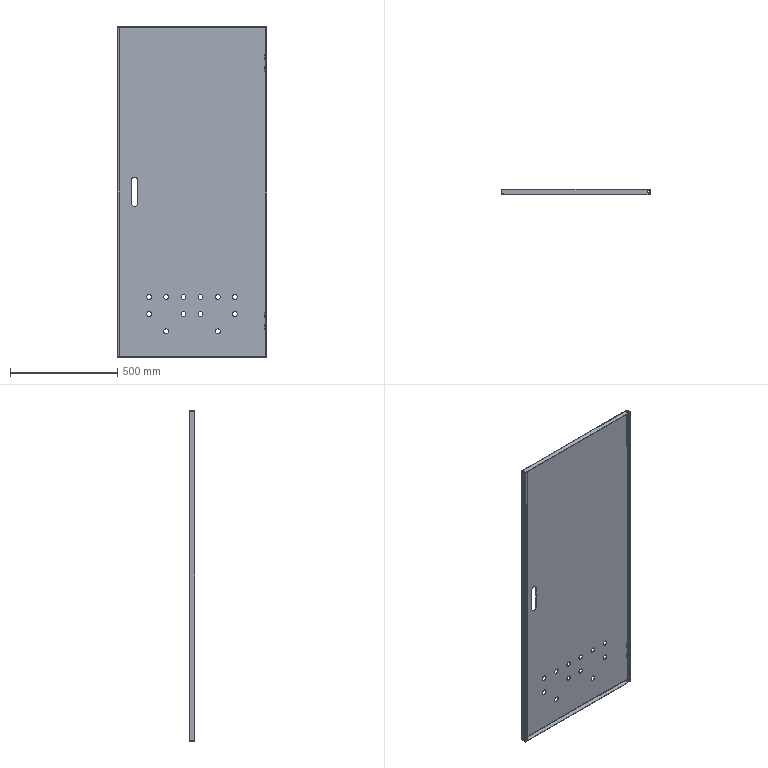Component | SolidWorks | OuterDoorAssembly1-1_OuterDoor1536X696-1 | 1 solid | 113 faces | volume 2347732 mm3 | plane 62 | cylinder 51 | commonest cylinder face diameters 22.5 x24 12.4 x8 5 x6 1 x6 12 x4 28 x3